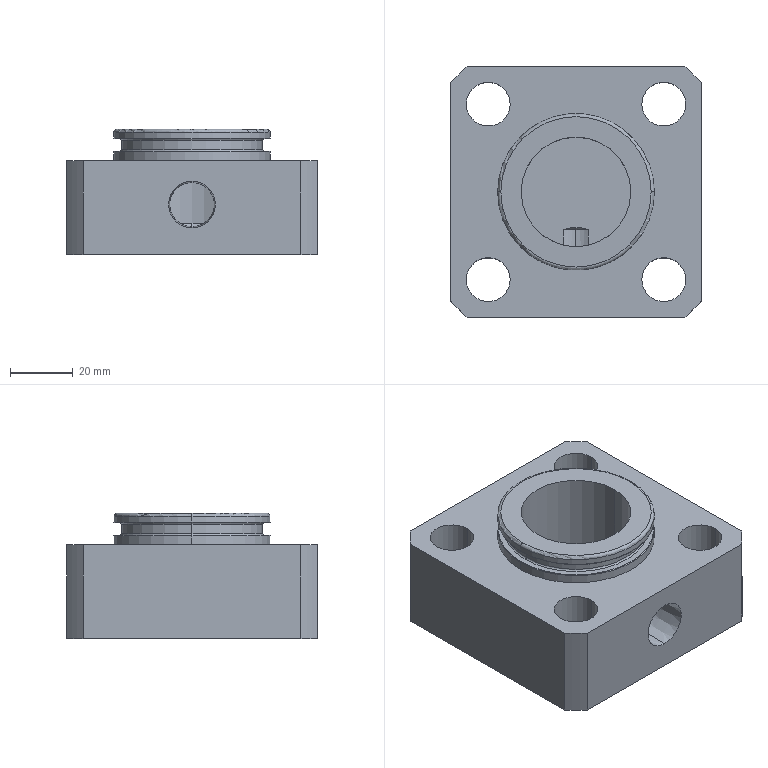Component | SolidWorks | Cylinder-1_RearEndCap-1 | 1 solid | 47 faces | volume 157437 mm3 | cylinder 22 | plane 11 | torus 10 | cone 4 | commonest cylinder face diameters 14 x8 50 x4 106 x4 45 x2 14.3 x2 35 x2